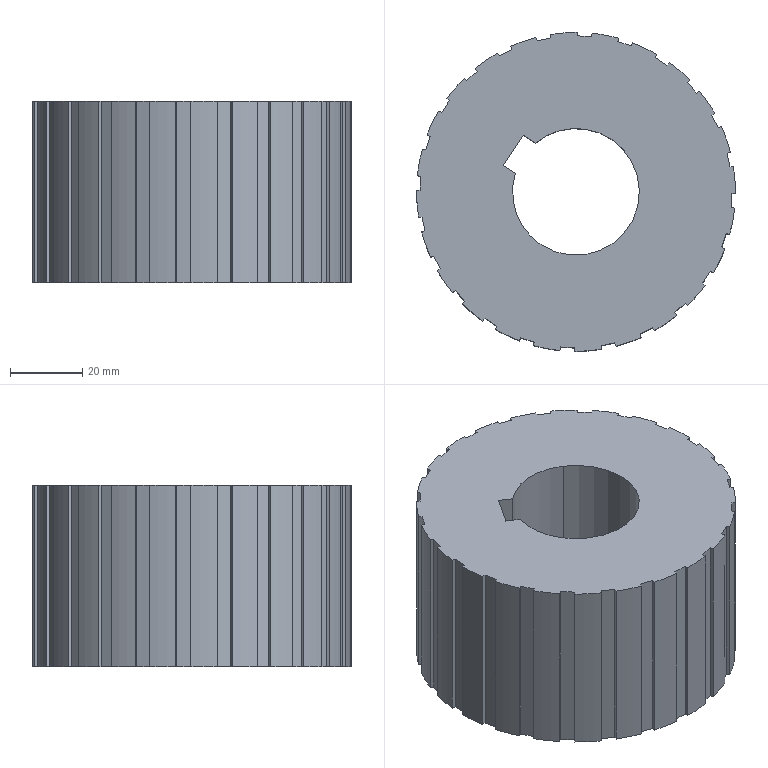Component | SolidWorks | NewTypeCurveBenderReinforcementFeedingWheel-DoubleWheel-1 | 1 solid | 107 faces | box 88 x 88 x 50 mm | volume 237333 mm3 | plane 78 | cylinder 29 | commonest cylinder face diameters 88 x24 35 x3 48 x2
build123d program:
from build123d import *

# Parameters (mm, degrees)
BOSS_EXTRUDE1_DEPTH = 50
CUT_EXTRUDE1_DEPTH  = 80.783
SKETCH4_R           = 24
CUT_EXTRUDE2_DEPTH  = 15


with BuildPart() as part:
    # Sketch1 → Boss-Extrude1 (new body)
    with BuildSketch(Plane.XY):
        with BuildLine():
            Line((-1.82, 43.962), (-1.65, 43))
            Line((-1.65, 43), (2.176, 43))
            Line((2.176, 43), (2.341, 43.938))
            ThreePointArc((2.341, 43.938), (6.002, 43.589), (9.62, 42.935))
            Line((9.62, 42.935), (9.535, 41.962))
            Line((9.535, 41.962), (13.231, 40.972))
            Line((13.231, 40.972), (13.633, 41.835))
            ThreePointArc((13.633, 41.835), (17.079, 40.55), (20.405, 38.982))
            Line((20.405, 38.982), (20.071, 38.064))
            Line((20.071, 38.064), (23.384, 36.151))
            Line((23.384, 36.151), (23.996, 36.88))
            ThreePointArc((23.996, 36.88), (26.992, 34.748), (29.799, 32.373))
            Line((29.799, 32.373), (29.239, 31.572))
            Line((29.239, 31.572), (31.944, 28.867))
            Line((31.944, 28.867), (32.724, 29.413))
            ThreePointArc((32.724, 29.413), (35.066, 26.578), (37.163, 23.557))
            Line((37.163, 23.557), (36.414, 22.929))
            Line((36.414, 22.929), (38.327, 19.616))
            Line((38.327, 19.616), (39.222, 19.941))
            ThreePointArc((39.222, 19.941), (40.75, 16.597), (41.993, 13.136))
            Line((41.993, 13.136), (41.108, 12.723))
            Line((41.108, 12.723), (42.098, 9.027))
            Line((42.098, 9.027), (43.046, 9.11))
            ThreePointArc((43.046, 9.11), (43.657, 5.484), (43.962, 1.82))
            Line((43.962, 1.82), (43, 1.65))
            Line((43, 1.65), (43, -2.176))
            Line((43, -2.176), (43.938, -2.341))
            ThreePointArc((43.938, -2.341), (43.589, -6.002), (42.935, -9.62))
            Line((42.935, -9.62), (41.962, -9.535))
            Line((41.962, -9.535), (40.972, -13.231))
            Line((40.972, -13.231), (41.835, -13.633))
            ThreePointArc((41.835, -13.633), (40.55, -17.079), (38.982, -20.405))
            Line((38.982, -20.405), (38.064, -20.071))
            Line((38.064, -20.071), (36.151, -23.384))
            Line((36.151, -23.384), (36.88, -23.996))
            ThreePointArc((36.88, -23.996), (34.748, -26.992), (32.373, -29.799))
            Line((32.373, -29.799), (31.572, -29.239))
            Line((31.572, -29.239), (28.867, -31.944))
            Line((28.867, -31.944), (29.413, -32.724))
            ThreePointArc((29.413, -32.724), (26.578, -35.066), (23.557, -37.163))
            Line((23.557, -37.163), (22.929, -36.414))
            Line((22.929, -36.414), (19.616, -38.327))
            Line((19.616, -38.327), (19.941, -39.222))
            ThreePointArc((19.941, -39.222), (16.597, -40.75), (13.136, -41.993))
            Line((13.136, -41.993), (12.723, -41.108))
            Line((12.723, -41.108), (9.027, -42.098))
            Line((9.027, -42.098), (9.11, -43.046))
            ThreePointArc((9.11, -43.046), (5.484, -43.657), (1.82, -43.962))
            Line((1.82, -43.962), (1.65, -43))
            Line((1.65, -43), (-2.176, -43))
            Line((-2.176, -43), (-2.341, -43.938))
            ThreePointArc((-2.341, -43.938), (-6.002, -43.589), (-9.62, -42.935))
            Line((-9.62, -42.935), (-9.535, -41.962))
            Line((-9.535, -41.962), (-13.231, -40.972))
            Line((-13.231, -40.972), (-13.633, -41.835))
            ThreePointArc((-13.633, -41.835), (-17.079, -40.55), (-20.405, -38.982))
            Line((-20.405, -38.982), (-20.071, -38.064))
            Line((-20.071, -38.064), (-23.384, -36.151))
            Line((-23.384, -36.151), (-23.996, -36.88))
            ThreePointArc((-23.996, -36.88), (-26.992, -34.748), (-29.799, -32.373))
            Line((-29.799, -32.373), (-29.239, -31.572))
            Line((-29.239, -31.572), (-31.944, -28.867))
            Line((-31.944, -28.867), (-32.724, -29.413))
            ThreePointArc((-32.724, -29.413), (-35.066, -26.578), (-37.163, -23.557))
            Line((-37.163, -23.557), (-36.414, -22.929))
            Line((-36.414, -22.929), (-38.327, -19.616))
            Line((-38.327, -19.616), (-39.222, -19.941))
            ThreePointArc((-39.222, -19.941), (-40.75, -16.597), (-41.993, -13.136))
            Line((-41.993, -13.136), (-41.108, -12.723))
            Line((-41.108, -12.723), (-42.098, -9.027))
            Line((-42.098, -9.027), (-43.046, -9.11))
            ThreePointArc((-43.046, -9.11), (-43.657, -5.484), (-43.962, -1.82))
            Line((-43.962, -1.82), (-43, -1.65))
            Line((-43, -1.65), (-43, 2.176))
            Line((-43, 2.176), (-43.938, 2.341))
            ThreePointArc((-43.938, 2.341), (-43.589, 6.002), (-42.935, 9.62))
            Line((-42.935, 9.62), (-41.962, 9.535))
            Line((-41.962, 9.535), (-40.972, 13.231))
            Line((-40.972, 13.231), (-41.835, 13.633))
            ThreePointArc((-41.835, 13.633), (-40.55, 17.079), (-38.982, 20.405))
            Line((-38.982, 20.405), (-38.064, 20.071))
            Line((-38.064, 20.071), (-36.151, 23.384))
            Line((-36.151, 23.384), (-36.88, 23.996))
            ThreePointArc((-36.88, 23.996), (-34.748, 26.992), (-32.373, 29.799))
            Line((-32.373, 29.799), (-31.572, 29.239))
            Line((-31.572, 29.239), (-28.867, 31.944))
            Line((-28.867, 31.944), (-29.413, 32.724))
            ThreePointArc((-29.413, 32.724), (-26.578, 35.066), (-23.557, 37.163))
            Line((-23.557, 37.163), (-22.929, 36.414))
            Line((-22.929, 36.414), (-19.616, 38.327))
            Line((-19.616, 38.327), (-19.941, 39.222))
            ThreePointArc((-19.941, 39.222), (-16.597, 40.75), (-13.136, 41.993))
            Line((-13.136, 41.993), (-12.723, 41.108))
            Line((-12.723, 41.108), (-9.027, 42.098))
            Line((-9.027, 42.098), (-9.11, 43.046))
            ThreePointArc((-9.11, 43.046), (-5.484, 43.657), (-1.82, 43.962))
        make_face()
    extrude(amount=BOSS_EXTRUDE1_DEPTH)

    # Sketch3 → Cut-Extrude1 (cut, through all)
    with BuildSketch(Plane(origin=(0, 0, 0), x_dir=(-1, 0, 0), z_dir=(0, 0, -1))):
        with BuildLine():
            Line((-5, 20.8), (5, 20.8))
            Line((5, 20.8), (5, 16.771))
            ThreePointArc((5, 16.771), (0, -17.5), (-5, 16.771))
            Line((-5, 16.771), (-5, 20.8))
        make_face()
    extrude(amount=-CUT_EXTRUDE1_DEPTH, mode=Mode.SUBTRACT)

    # Sketch4 → Cut-Extrude2 (cut)
    with BuildSketch(Plane.XY.offset(50)):
        Circle(SKETCH4_R)
    extrude(amount=-CUT_EXTRUDE2_DEPTH, mode=Mode.SUBTRACT)


solid = part.part

# Placed as in the assembly
solid = solid.moved(Location((50, -88, -119), (180, 0, 123.489)))